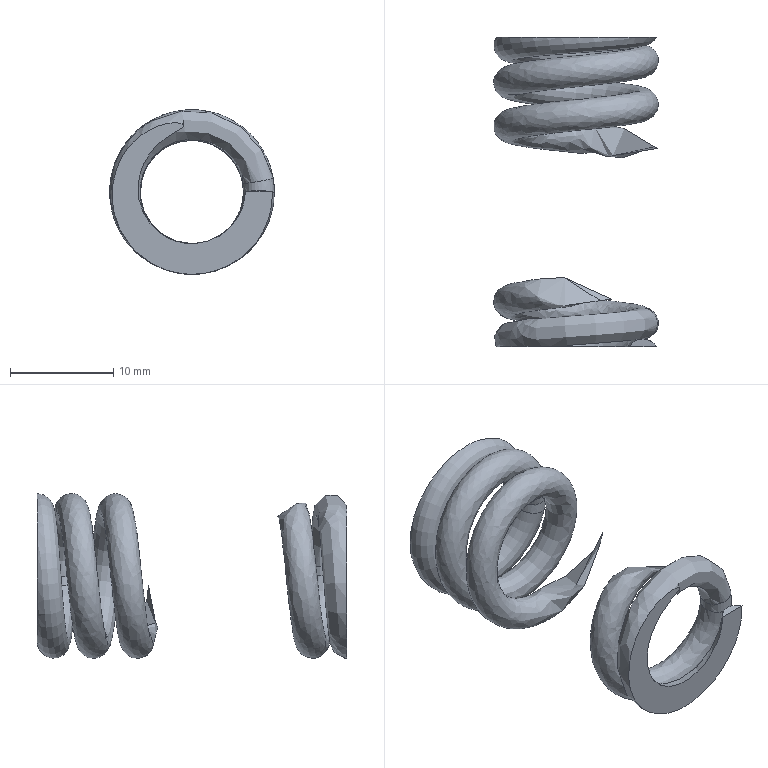Component | NX | SPRING | 1 solid | 9 faces | volume 2161 mm3 | spline 5 | plane 4